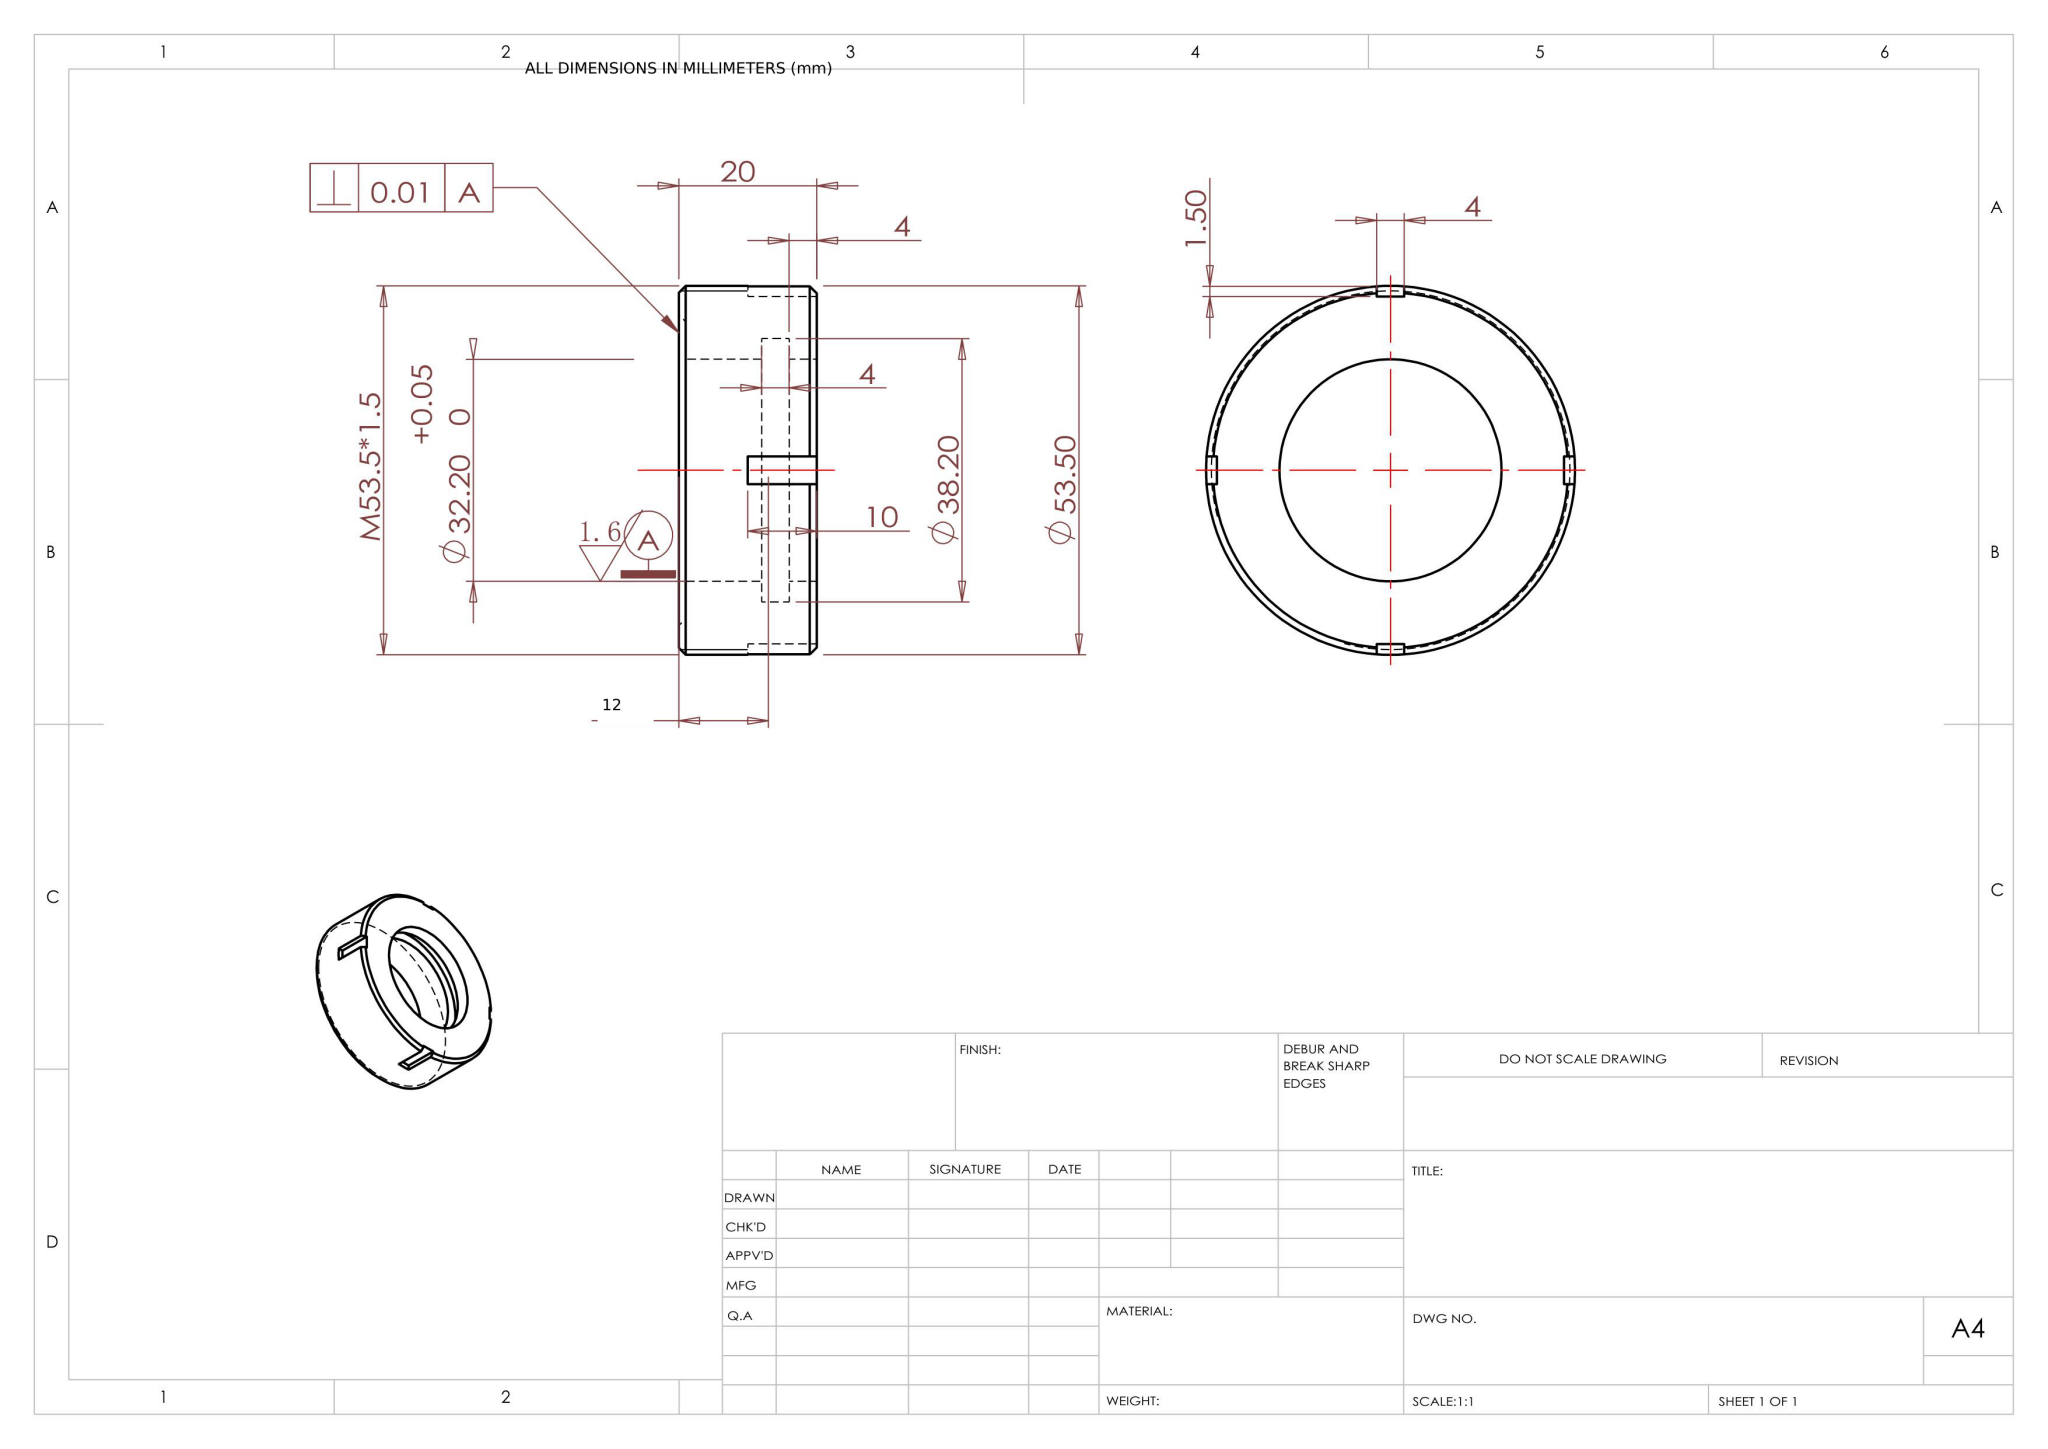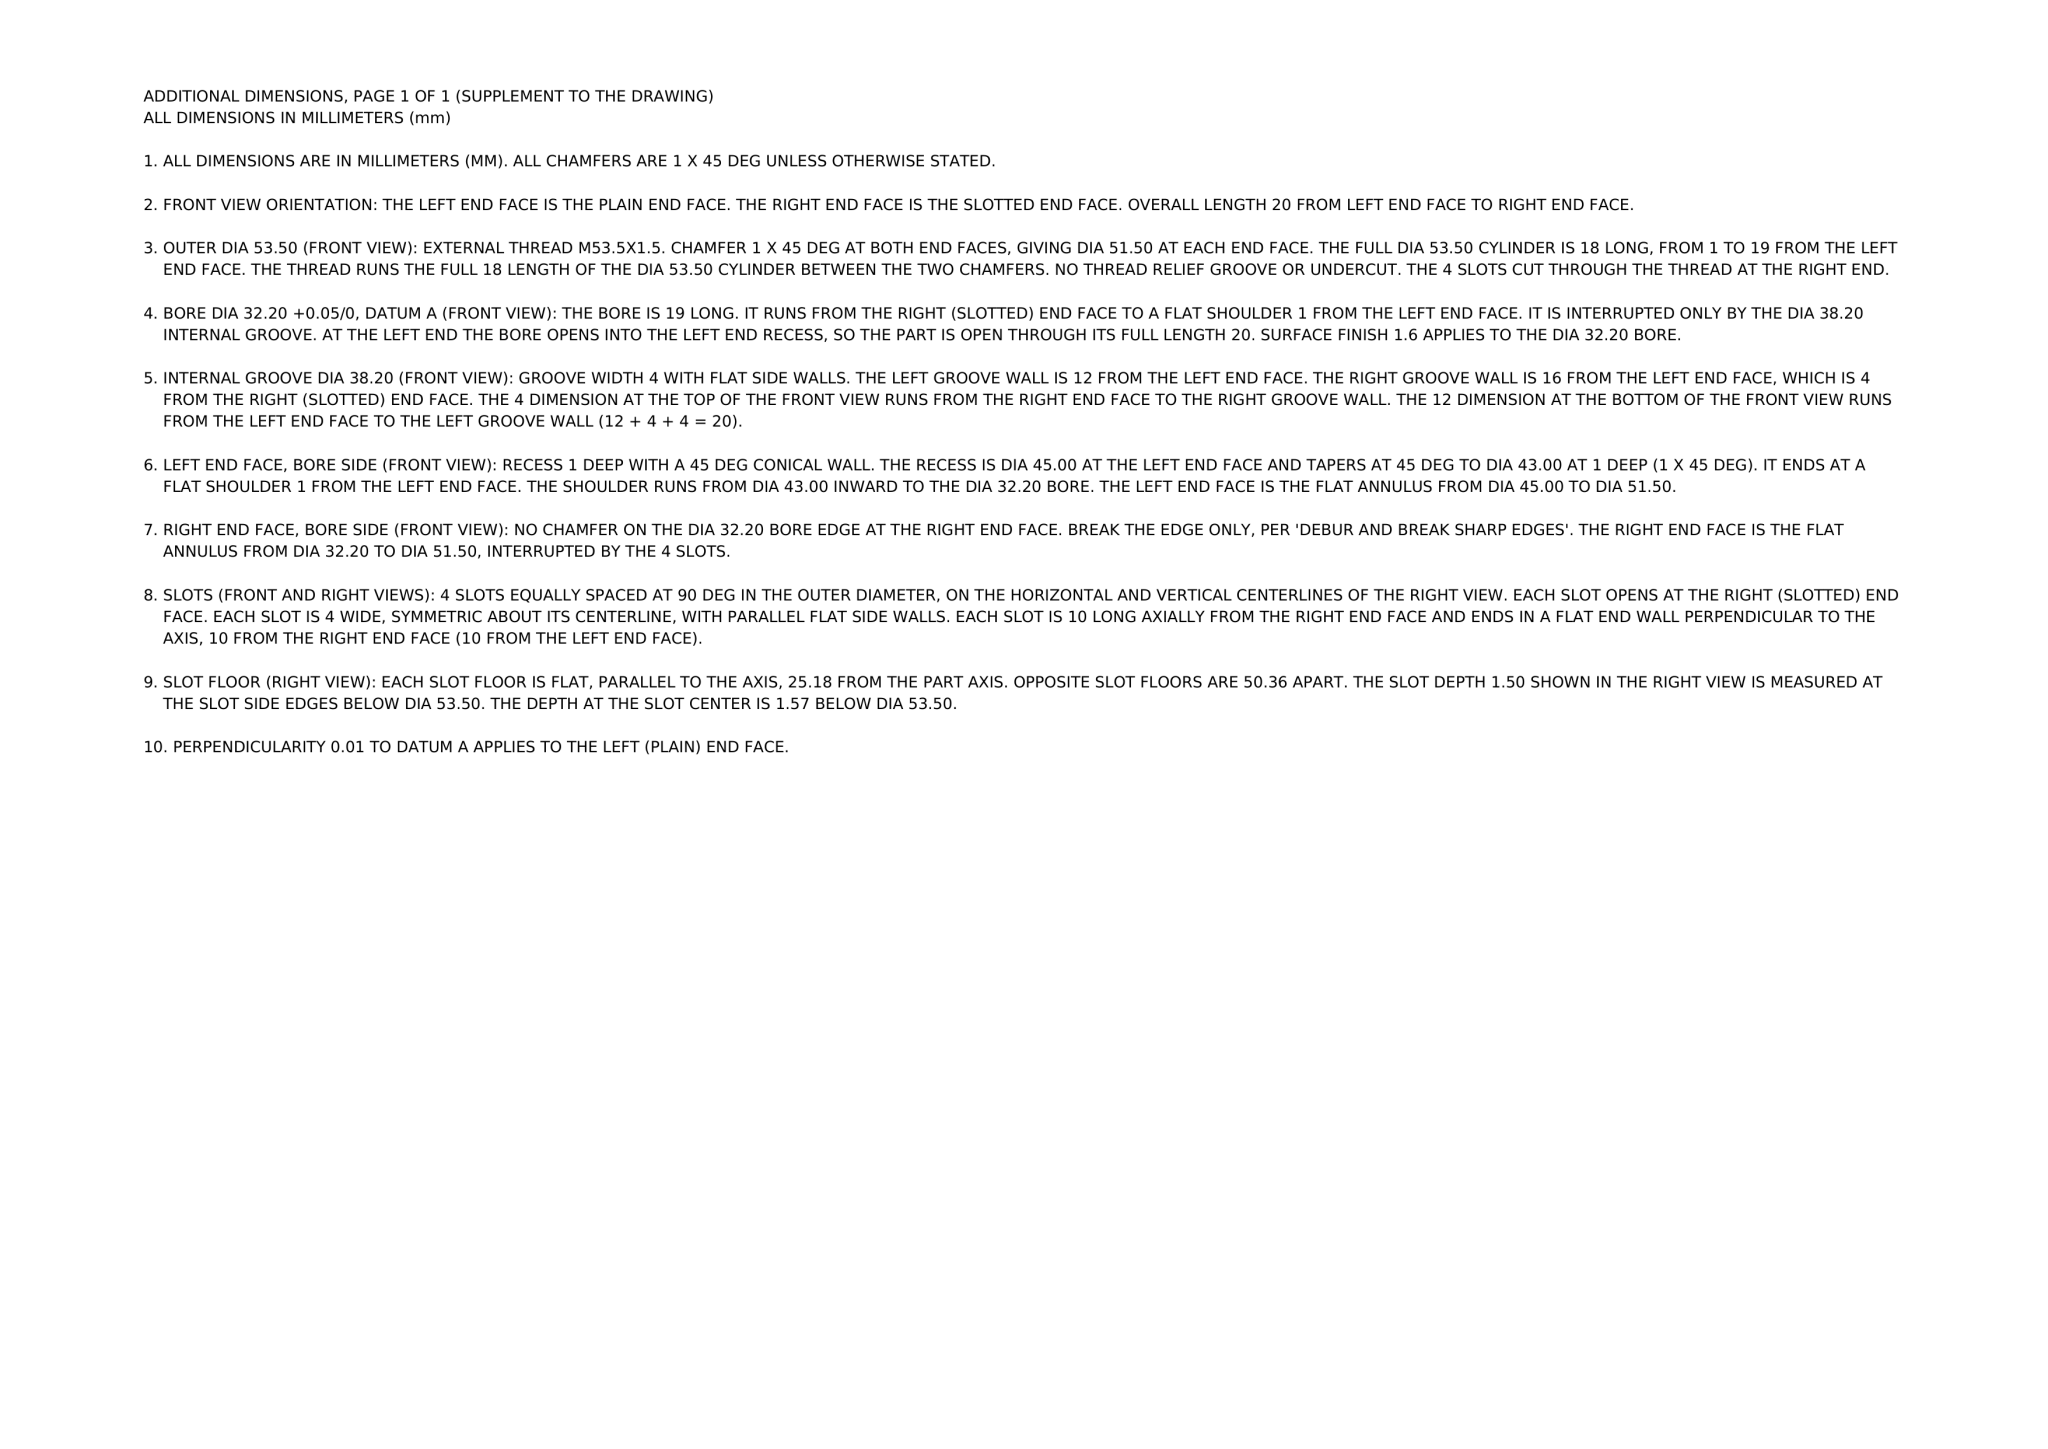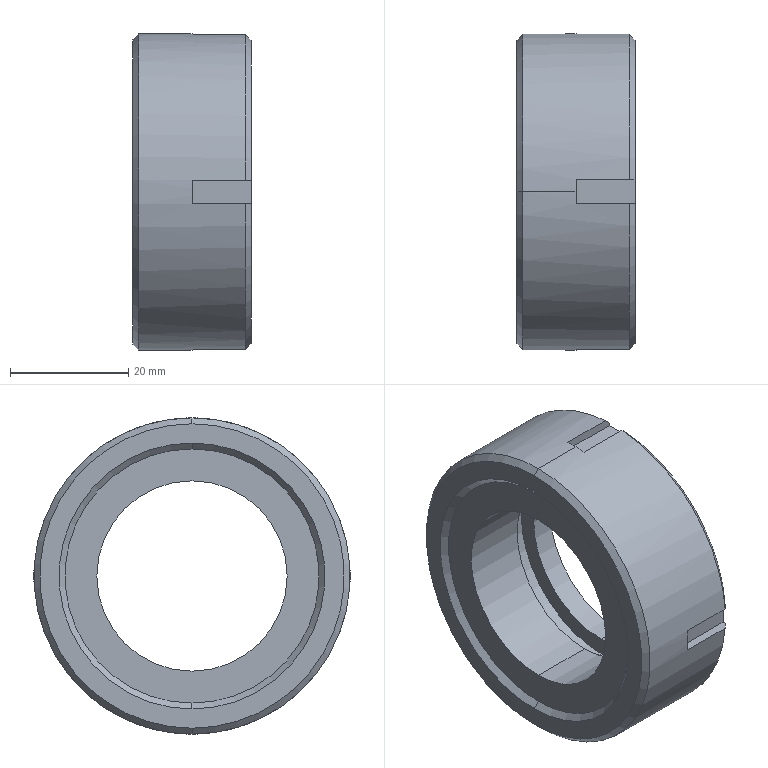Part | NX | mm | 1 solid | 37 faces | box 20 x 53.5 x 53.5 mm | volume 26234 mm3 | plane 21 | cone 8 | cylinder 8 | commonest cylinder face diameters 32.2 x4 53.5 x2 38.2 x2